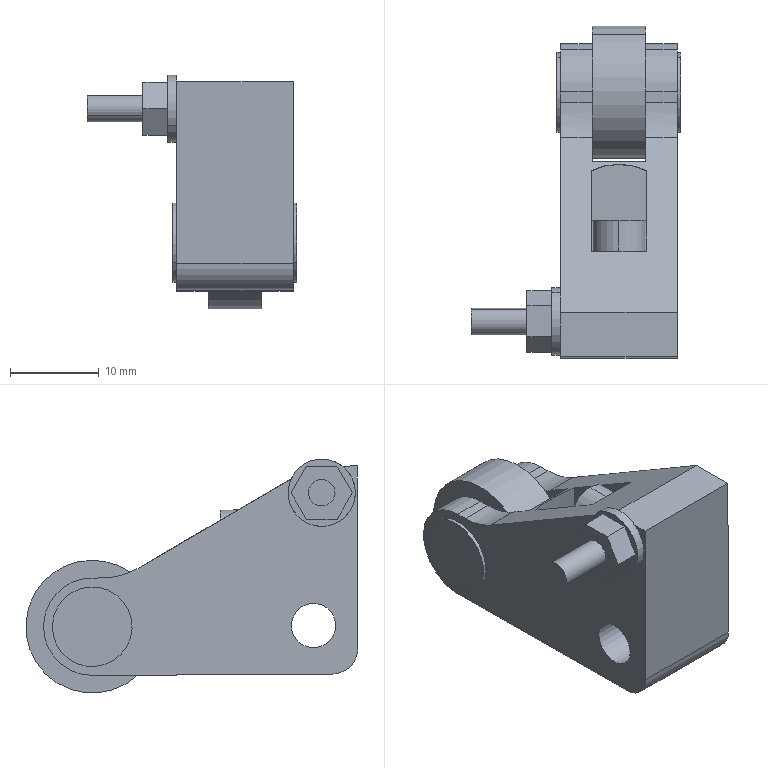Component | SolidWorks | RSDQA32-20DD-M9BL(0_0)-1_RSQ32-20D_LEVER-1 | 1 solid | 59 faces | volume 7464 mm3 | plane 37 | cylinder 22 | commonest cylinder face diameters 11 x4 9 x4 6 x3 5 x2 7.6 x2 15 x2 3 x2 16 x2